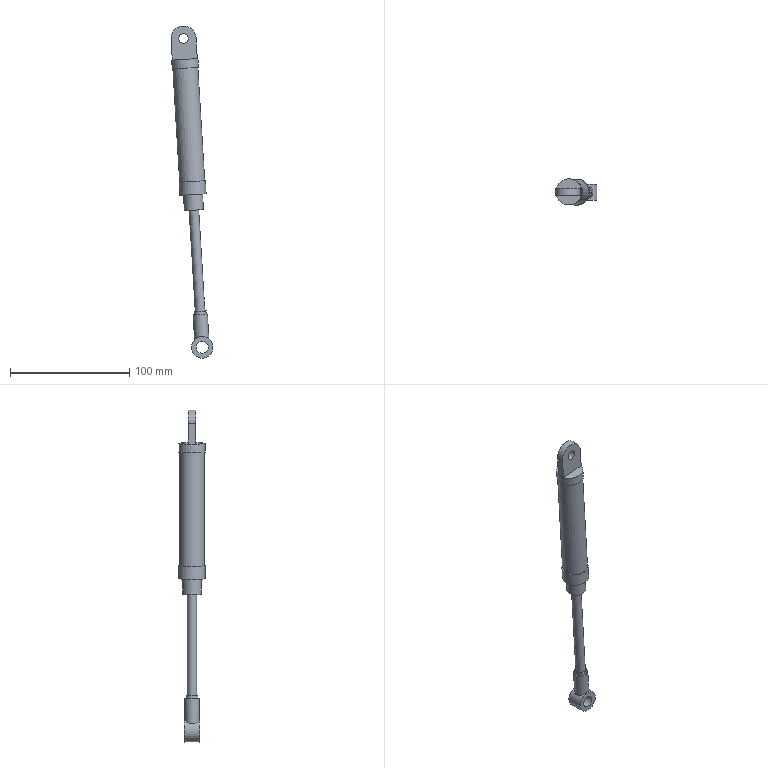Component | NX | CYLINDER | 4 solids | 28 faces | volume 52018 mm3 | plane 16 | cylinder 12 | commonest cylinder face diameters 8 x3 22 x2 21 x2 10 x2 16 x1 18 x1 12 x1